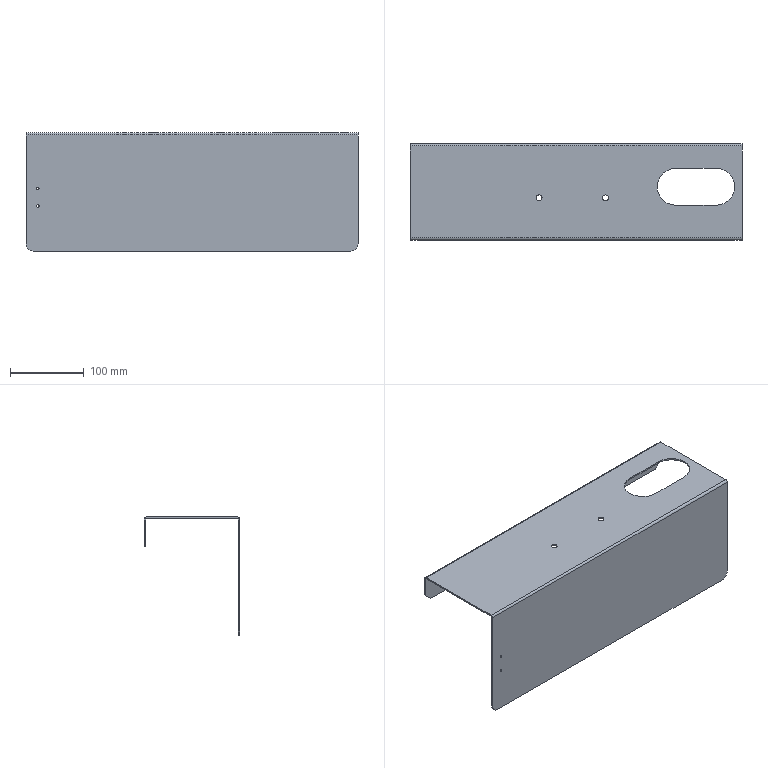Component | SolidWorks | -LowerGuard-1 | 1 solid | 39 faces | box 450 x 130 x 160 mm | volume 282110 mm3 | plane 22 | cylinder 17 | commonest cylinder face diameters 3.3 x4 8 x4 50 x3 5.473 x2 1.473 x2 20 x2
STEP:
#1=COLOUR_RGB('',0.7922,0.8196,0.9333);
#2=FILL_AREA_STYLE_COLOUR('',#1);
#3=FILL_AREA_STYLE('',(#2));
#4=SURFACE_STYLE_FILL_AREA(#3);
#5=SURFACE_SIDE_STYLE('',(#4));
#6=SURFACE_STYLE_USAGE(.BOTH.,#5);
#7=PRESENTATION_STYLE_ASSIGNMENT((#6));
#8=CARTESIAN_POINT('',(9.843,43.091,6.89));
#9=VERTEX_POINT('',#8);
#10=CARTESIAN_POINT('',(8.858,44.075,6.89));
#11=VERTEX_POINT('',#10);
#12=CARTESIAN_POINT('',(8.858,43.091,6.89));
#13=DIRECTION('',(-0.,0.,1.));
#14=DIRECTION('',(1.,0.,0.));
#15=AXIS2_PLACEMENT_3D('',#12,#13,#14);
#16=CIRCLE('',#15,0.9843);
#17=EDGE_CURVE('',#9,#11,#16,.T.);
#18=ORIENTED_EDGE('',*,*,#17,.F.);
#19=CARTESIAN_POINT('',(9.843,43.091,6.969));
#20=VERTEX_POINT('',#19);
#21=CARTESIAN_POINT('',(9.843,43.091,0.6693));
#22=DIRECTION('',(-0.,0.,1.));
#23=VECTOR('',#22,39.37);
#24=LINE('',#21,#23);
#25=EDGE_CURVE('',#9,#20,#24,.T.);
#26=ORIENTED_EDGE('',*,*,#25,.T.);
#27=CARTESIAN_POINT('',(8.858,44.075,6.969));
#28=VERTEX_POINT('',#27);
#29=CARTESIAN_POINT('',(8.858,43.091,6.969));
#30=DIRECTION('',(-0.,0.,1.));
#31=DIRECTION('',(1.,0.,0.));
#32=AXIS2_PLACEMENT_3D('',#29,#30,#31);
#33=CIRCLE('',#32,0.9843);
#34=EDGE_CURVE('',#20,#28,#33,.T.);
#35=ORIENTED_EDGE('',*,*,#34,.T.);
#36=CARTESIAN_POINT('',(8.858,44.075,0.6693));
#37=DIRECTION('',(-0.,0.,1.));
#38=VECTOR('',#37,39.37);
#39=LINE('',#36,#38);
#40=EDGE_CURVE('',#11,#28,#39,.T.);
#41=ORIENTED_EDGE('',*,*,#40,.F.);
#42=EDGE_LOOP('',(#18,#26,#35,#41));
#43=FACE_OUTER_BOUND('',#42,.T.);
#44=CARTESIAN_POINT('',(8.858,43.091,0.6693));
#45=DIRECTION('',(-0.,0.,1.));
#46=DIRECTION('',(1.,0.,0.));
#47=AXIS2_PLACEMENT_3D('',#44,#45,#46);
#48=CYLINDRICAL_SURFACE('',#47,0.9843);
#49=ADVANCED_FACE('',(#43),#48,.F.);
#50=CARTESIAN_POINT('',(-6.85,40.256,4.081));
#51=VERTEX_POINT('',#50);
#52=CARTESIAN_POINT('',(-6.85,40.256,3.951));
#53=VERTEX_POINT('',#52);
#54=CARTESIAN_POINT('',(-6.85,40.256,4.016));
#55=DIRECTION('',(-0.,1.,-0.));
#56=DIRECTION('',(0.,0.,-1.));
#57=AXIS2_PLACEMENT_3D('',#54,#55,#56);
#58=CIRCLE('',#57,0.06496);
#59=EDGE_CURVE('',#51,#53,#58,.T.);
#60=ORIENTED_EDGE('',*,*,#59,.F.);
#61=CARTESIAN_POINT('',(-6.85,40.335,4.081));
#62=VERTEX_POINT('',#61);
#63=CARTESIAN_POINT('',(-6.85,40.335,4.081));
#64=DIRECTION('',(-0.,1.,-0.));
#65=VECTOR('',#64,39.37);
#66=LINE('',#63,#65);
#67=EDGE_CURVE('',#51,#62,#66,.T.);
#68=ORIENTED_EDGE('',*,*,#67,.T.);
#69=CARTESIAN_POINT('',(-6.85,40.335,3.951));
#70=VERTEX_POINT('',#69);
#71=CARTESIAN_POINT('',(-6.85,40.335,4.016));
#72=DIRECTION('',(-0.,1.,-0.));
#73=DIRECTION('',(0.,0.,-1.));
#74=AXIS2_PLACEMENT_3D('',#71,#72,#73);
#75=CIRCLE('',#74,0.06496);
#76=EDGE_CURVE('',#62,#70,#75,.T.);
#77=ORIENTED_EDGE('',*,*,#76,.T.);
#78=CARTESIAN_POINT('',(-6.85,40.335,3.951));
#79=DIRECTION('',(-0.,1.,-0.));
#80=VECTOR('',#79,39.37);
#81=LINE('',#78,#80);
#82=EDGE_CURVE('',#53,#70,#81,.T.);
#83=ORIENTED_EDGE('',*,*,#82,.F.);
#84=EDGE_LOOP('',(#60,#68,#77,#83));
#85=FACE_OUTER_BOUND('',#84,.T.);
#86=CARTESIAN_POINT('',(-6.85,40.335,4.016));
#87=DIRECTION('',(-0.,1.,-0.));
#88=DIRECTION('',(0.,0.,-1.));
#89=AXIS2_PLACEMENT_3D('',#86,#87,#88);
#90=CYLINDRICAL_SURFACE('',#89,0.06496);
#91=ADVANCED_FACE('',(#85),#90,.F.);
#92=CARTESIAN_POINT('',(-6.85,40.256,3.136));
#93=VERTEX_POINT('',#92);
#94=CARTESIAN_POINT('',(-6.85,40.256,3.006));
#95=VERTEX_POINT('',#94);
#96=CARTESIAN_POINT('',(-6.85,40.256,3.071));
#97=DIRECTION('',(-0.,1.,-0.));
#98=DIRECTION('',(0.,0.,-1.));
#99=AXIS2_PLACEMENT_3D('',#96,#97,#98);
#100=CIRCLE('',#99,0.06496);
#101=EDGE_CURVE('',#93,#95,#100,.T.);
#102=ORIENTED_EDGE('',*,*,#101,.F.);
#103=CARTESIAN_POINT('',(-6.85,40.335,3.136));
#104=VERTEX_POINT('',#103);
#105=CARTESIAN_POINT('',(-6.85,40.335,3.136));
#106=DIRECTION('',(-0.,1.,-0.));
#107=VECTOR('',#106,39.37);
#108=LINE('',#105,#107);
#109=EDGE_CURVE('',#93,#104,#108,.T.);
#110=ORIENTED_EDGE('',*,*,#109,.T.);
#111=CARTESIAN_POINT('',(-6.85,40.335,3.006));
#112=VERTEX_POINT('',#111);
#113=CARTESIAN_POINT('',(-6.85,40.335,3.071));
#114=DIRECTION('',(-0.,1.,-0.));
#115=DIRECTION('',(0.,0.,-1.));
#116=AXIS2_PLACEMENT_3D('',#113,#114,#115);
#117=CIRCLE('',#116,0.06496);
#118=EDGE_CURVE('',#104,#112,#117,.T.);
#119=ORIENTED_EDGE('',*,*,#118,.T.);
#120=CARTESIAN_POINT('',(-6.85,40.335,3.006));
#121=DIRECTION('',(-0.,1.,-0.));
#122=VECTOR('',#121,39.37);
#123=LINE('',#120,#122);
#124=EDGE_CURVE('',#95,#112,#123,.T.);
#125=ORIENTED_EDGE('',*,*,#124,.F.);
#126=EDGE_LOOP('',(#102,#110,#119,#125));
#127=FACE_OUTER_BOUND('',#126,.T.);
#128=CARTESIAN_POINT('',(-6.85,40.335,3.071));
#129=DIRECTION('',(-0.,1.,-0.));
#130=DIRECTION('',(0.,0.,-1.));
#131=AXIS2_PLACEMENT_3D('',#128,#129,#130);
#132=CYLINDRICAL_SURFACE('',#131,0.06496);
#133=ADVANCED_FACE('',(#127),#132,.F.);
#134=CARTESIAN_POINT('',(2.795,42.5,6.89));
#135=VERTEX_POINT('',#134);
#136=CARTESIAN_POINT('',(3.11,42.5,6.89));
#137=VERTEX_POINT('',#136);
#138=CARTESIAN_POINT('',(2.953,42.5,6.89));
#139=DIRECTION('',(-0.,0.,1.));
#140=DIRECTION('',(1.,0.,0.));
#141=AXIS2_PLACEMENT_3D('',#138,#139,#140);
#142=CIRCLE('',#141,0.1575);
#143=EDGE_CURVE('',#135,#137,#142,.T.);
#144=ORIENTED_EDGE('',*,*,#143,.F.);
#145=CARTESIAN_POINT('',(2.795,42.5,6.969));
#146=VERTEX_POINT('',#145);
#147=CARTESIAN_POINT('',(2.795,42.5,6.575));
#148=DIRECTION('',(-0.,0.,1.));
#149=VECTOR('',#148,39.37);
#150=LINE('',#147,#149);
#151=EDGE_CURVE('',#135,#146,#150,.T.);
#152=ORIENTED_EDGE('',*,*,#151,.T.);
#153=CARTESIAN_POINT('',(3.11,42.5,6.969));
#154=VERTEX_POINT('',#153);
#155=CARTESIAN_POINT('',(2.953,42.5,6.969));
#156=DIRECTION('',(-0.,0.,1.));
#157=DIRECTION('',(1.,0.,0.));
#158=AXIS2_PLACEMENT_3D('',#155,#156,#157);
#159=CIRCLE('',#158,0.1575);
#160=EDGE_CURVE('',#146,#154,#159,.T.);
#161=ORIENTED_EDGE('',*,*,#160,.T.);
#162=CARTESIAN_POINT('',(3.11,42.5,6.575));
#163=DIRECTION('',(-0.,0.,1.));
#164=VECTOR('',#163,39.37);
#165=LINE('',#162,#164);
#166=EDGE_CURVE('',#137,#154,#165,.T.);
#167=ORIENTED_EDGE('',*,*,#166,.F.);
#168=EDGE_LOOP('',(#144,#152,#161,#167));
#169=FACE_OUTER_BOUND('',#168,.T.);
#170=CARTESIAN_POINT('',(2.953,42.5,6.575));
#171=DIRECTION('',(-0.,0.,1.));
#172=DIRECTION('',(1.,0.,0.));
#173=AXIS2_PLACEMENT_3D('',#170,#171,#172);
#174=CYLINDRICAL_SURFACE('',#173,0.1575);
#175=ADVANCED_FACE('',(#169),#174,.F.);
#176=CARTESIAN_POINT('',(-0.748,42.5,6.89));
#177=VERTEX_POINT('',#176);
#178=CARTESIAN_POINT('',(-0.4331,42.5,6.89));
#179=VERTEX_POINT('',#178);
#180=CARTESIAN_POINT('',(-0.5906,42.5,6.89));
#181=DIRECTION('',(-0.,0.,1.));
#182=DIRECTION('',(1.,0.,0.));
#183=AXIS2_PLACEMENT_3D('',#180,#181,#182);
#184=CIRCLE('',#183,0.1575);
#185=EDGE_CURVE('',#177,#179,#184,.T.);
#186=ORIENTED_EDGE('',*,*,#185,.F.);
#187=CARTESIAN_POINT('',(-0.748,42.5,6.969));
#188=VERTEX_POINT('',#187);
#189=CARTESIAN_POINT('',(-0.748,42.5,6.575));
#190=DIRECTION('',(-0.,0.,1.));
#191=VECTOR('',#190,39.37);
#192=LINE('',#189,#191);
#193=EDGE_CURVE('',#177,#188,#192,.T.);
#194=ORIENTED_EDGE('',*,*,#193,.T.);
#195=CARTESIAN_POINT('',(-0.4331,42.5,6.969));
#196=VERTEX_POINT('',#195);
#197=CARTESIAN_POINT('',(-0.5906,42.5,6.969));
#198=DIRECTION('',(-0.,0.,1.));
#199=DIRECTION('',(1.,0.,0.));
#200=AXIS2_PLACEMENT_3D('',#197,#198,#199);
#201=CIRCLE('',#200,0.1575);
#202=EDGE_CURVE('',#188,#196,#201,.T.);
#203=ORIENTED_EDGE('',*,*,#202,.T.);
#204=CARTESIAN_POINT('',(-0.4331,42.5,6.575));
#205=DIRECTION('',(-0.,0.,1.));
#206=VECTOR('',#205,39.37);
#207=LINE('',#204,#206);
#208=EDGE_CURVE('',#179,#196,#207,.T.);
#209=ORIENTED_EDGE('',*,*,#208,.F.);
#210=EDGE_LOOP('',(#186,#194,#203,#209));
#211=FACE_OUTER_BOUND('',#210,.T.);
#212=CARTESIAN_POINT('',(-0.5906,42.5,6.575));
#213=DIRECTION('',(-0.,0.,1.));
#214=DIRECTION('',(1.,0.,0.));
#215=AXIS2_PLACEMENT_3D('',#212,#213,#214);
#216=CYLINDRICAL_SURFACE('',#215,0.1575);
#217=ADVANCED_FACE('',(#211),#216,.F.);
#218=CARTESIAN_POINT('',(-7.48,40.256,6.861));
#219=VERTEX_POINT('',#218);
#220=CARTESIAN_POINT('',(-7.48,40.335,6.861));
#221=VERTEX_POINT('',#220);
#222=CARTESIAN_POINT('',(-7.48,40.256,6.861));
#223=DIRECTION('',(-0.,1.,-0.));
#224=VECTOR('',#223,39.37);
#225=LINE('',#222,#224);
#226=EDGE_CURVE('',#219,#221,#225,.T.);
#227=ORIENTED_EDGE('',*,*,#226,.F.);
#228=CARTESIAN_POINT('',(-7.48,40.364,6.969));
#229=VERTEX_POINT('',#228);
#230=CARTESIAN_POINT('',(-7.48,40.364,6.861));
#231=DIRECTION('',(1.,0.,0.));
#232=DIRECTION('',(0.,0.,1.));
#233=AXIS2_PLACEMENT_3D('',#230,#231,#232);
#234=CIRCLE('',#233,0.1077);
#235=EDGE_CURVE('',#229,#219,#234,.T.);
#236=ORIENTED_EDGE('',*,*,#235,.F.);
#237=CARTESIAN_POINT('',(-7.48,40.364,6.89));
#238=VERTEX_POINT('',#237);
#239=CARTESIAN_POINT('',(-7.48,40.364,6.89));
#240=DIRECTION('',(-0.,0.,1.));
#241=VECTOR('',#240,39.37);
#242=LINE('',#239,#241);
#243=EDGE_CURVE('',#238,#229,#242,.T.);
#244=ORIENTED_EDGE('',*,*,#243,.F.);
#245=CARTESIAN_POINT('',(-7.48,40.364,6.861));
#246=DIRECTION('',(1.,0.,0.));
#247=DIRECTION('',(0.,0.,1.));
#248=AXIS2_PLACEMENT_3D('',#245,#246,#247);
#249=CIRCLE('',#248,0.029);
#250=EDGE_CURVE('',#238,#221,#249,.T.);
#251=ORIENTED_EDGE('',*,*,#250,.T.);
#252=EDGE_LOOP('',(#227,#236,#244,#251));
#253=FACE_OUTER_BOUND('',#252,.T.);
#254=CARTESIAN_POINT('',(-7.48,40.256,6.861));
#255=DIRECTION('',(-1.,-0.,-0.));
#256=DIRECTION('',(-0.,0.,1.));
#257=AXIS2_PLACEMENT_3D('',#254,#255,#256);
#258=PLANE('',#257);
#259=ADVANCED_FACE('',(#253),#258,.T.);
#260=CARTESIAN_POINT('',(-7.48,40.335,1.063));
#261=VERTEX_POINT('',#260);
#262=CARTESIAN_POINT('',(-7.48,40.335,6.969));
#263=DIRECTION('',(0.,-0.,-1.));
#264=VECTOR('',#263,39.37);
#265=LINE('',#262,#264);
#266=EDGE_CURVE('',#221,#261,#265,.T.);
#267=ORIENTED_EDGE('',*,*,#266,.T.);
#268=CARTESIAN_POINT('',(-7.48,40.256,1.063));
#269=VERTEX_POINT('',#268);
#270=CARTESIAN_POINT('',(-7.48,40.364,1.063));
#271=DIRECTION('',(0.,-1.,0.));
#272=VECTOR('',#271,39.37);
#273=LINE('',#270,#272);
#274=EDGE_CURVE('',#261,#269,#273,.T.);
#275=ORIENTED_EDGE('',*,*,#274,.T.);
#276=CARTESIAN_POINT('',(-7.48,40.256,6.969));
#277=DIRECTION('',(0.,-0.,-1.));
#278=VECTOR('',#277,39.37);
#279=LINE('',#276,#278);
#280=EDGE_CURVE('',#219,#269,#279,.T.);
#281=ORIENTED_EDGE('',*,*,#280,.F.);
#282=ORIENTED_EDGE('',*,*,#226,.T.);
#283=EDGE_LOOP('',(#267,#275,#281,#282));
#284=FACE_OUTER_BOUND('',#283,.T.);
#285=CARTESIAN_POINT('',(-7.48,40.364,6.89));
#286=DIRECTION('',(-1.,-0.,-0.));
#287=DIRECTION('',(-0.,0.,1.));
#288=AXIS2_PLACEMENT_3D('',#285,#286,#287);
#289=PLANE('',#288);
#290=ADVANCED_FACE('',(#284),#289,.T.);
#291=CARTESIAN_POINT('',(10.236,40.364,6.969));
#292=VERTEX_POINT('',#291);
#293=CARTESIAN_POINT('',(10.236,40.364,6.89));
#294=VERTEX_POINT('',#293);
#295=CARTESIAN_POINT('',(10.236,40.364,6.969));
#296=DIRECTION('',(0.,-0.,-1.));
#297=VECTOR('',#296,39.37);
#298=LINE('',#295,#297);
#299=EDGE_CURVE('',#292,#294,#298,.T.);
#300=ORIENTED_EDGE('',*,*,#299,.F.);
#301=CARTESIAN_POINT('',(10.236,40.256,6.861));
#302=VERTEX_POINT('',#301);
#303=CARTESIAN_POINT('',(10.236,40.364,6.861));
#304=DIRECTION('',(1.,0.,0.));
#305=DIRECTION('',(0.,0.,1.));
#306=AXIS2_PLACEMENT_3D('',#303,#304,#305);
#307=CIRCLE('',#306,0.1077);
#308=EDGE_CURVE('',#292,#302,#307,.T.);
#309=ORIENTED_EDGE('',*,*,#308,.T.);
#310=CARTESIAN_POINT('',(10.236,40.335,6.861));
#311=VERTEX_POINT('',#310);
#312=CARTESIAN_POINT('',(10.236,40.335,6.861));
#313=DIRECTION('',(0.,-1.,0.));
#314=VECTOR('',#313,39.37);
#315=LINE('',#312,#314);
#316=EDGE_CURVE('',#311,#302,#315,.T.);
#317=ORIENTED_EDGE('',*,*,#316,.F.);
#318=CARTESIAN_POINT('',(10.236,40.364,6.861));
#319=DIRECTION('',(1.,0.,0.));
#320=DIRECTION('',(0.,0.,1.));
#321=AXIS2_PLACEMENT_3D('',#318,#319,#320);
#322=CIRCLE('',#321,0.029);
#323=EDGE_CURVE('',#294,#311,#322,.T.);
#324=ORIENTED_EDGE('',*,*,#323,.F.);
#325=EDGE_LOOP('',(#300,#309,#317,#324));
#326=FACE_OUTER_BOUND('',#325,.T.);
#327=CARTESIAN_POINT('',(10.236,40.364,6.969));
#328=DIRECTION('',(1.,0.,0.));
#329=DIRECTION('',(0.,-0.,-1.));
#330=AXIS2_PLACEMENT_3D('',#327,#328,#329);
#331=PLANE('',#330);
#332=ADVANCED_FACE('',(#326),#331,.T.);
#333=CARTESIAN_POINT('',(10.236,45.266,6.969));
#334=VERTEX_POINT('',#333);
#335=CARTESIAN_POINT('',(10.236,45.177,6.969));
#336=DIRECTION('',(0.,-1.,0.));
#337=VECTOR('',#336,39.37);
#338=LINE('',#335,#337);
#339=EDGE_CURVE('',#334,#292,#338,.T.);
#340=ORIENTED_EDGE('',*,*,#339,.T.);
#341=ORIENTED_EDGE('',*,*,#299,.T.);
#342=CARTESIAN_POINT('',(10.236,45.266,6.89));
#343=VERTEX_POINT('',#342);
#344=CARTESIAN_POINT('',(10.236,45.177,6.89));
#345=DIRECTION('',(0.,-1.,0.));
#346=VECTOR('',#345,39.37);
#347=LINE('',#344,#346);
#348=EDGE_CURVE('',#343,#294,#347,.T.);
#349=ORIENTED_EDGE('',*,*,#348,.F.);
#350=CARTESIAN_POINT('',(10.236,45.266,6.89));
#351=DIRECTION('',(-0.,0.,1.));
#352=VECTOR('',#351,39.37);
#353=LINE('',#350,#352);
#354=EDGE_CURVE('',#343,#334,#353,.T.);
#355=ORIENTED_EDGE('',*,*,#354,.T.);
#356=EDGE_LOOP('',(#340,#341,#349,#355));
#357=FACE_OUTER_BOUND('',#356,.T.);
#358=CARTESIAN_POINT('',(10.236,40.335,6.861));
#359=DIRECTION('',(1.,0.,0.));
#360=DIRECTION('',(0.,-0.,-1.));
#361=AXIS2_PLACEMENT_3D('',#358,#359,#360);
#362=PLANE('',#361);
#363=ADVANCED_FACE('',(#357),#362,.T.);
#364=CARTESIAN_POINT('',(-6.85,40.335,4.016));
#365=DIRECTION('',(-0.,1.,-0.));
#366=DIRECTION('',(0.,0.,-1.));
#367=AXIS2_PLACEMENT_3D('',#364,#365,#366);
#368=CIRCLE('',#367,0.06496);
#369=EDGE_CURVE('',#70,#62,#368,.T.);
#370=ORIENTED_EDGE('',*,*,#369,.F.);
#371=ORIENTED_EDGE('',*,*,#76,.F.);
#372=EDGE_LOOP('',(#370,#371));
#373=FACE_BOUND('',#372,.T.);
#374=CARTESIAN_POINT('',(-6.85,40.335,3.071));
#375=DIRECTION('',(-0.,1.,-0.));
#376=DIRECTION('',(0.,0.,-1.));
#377=AXIS2_PLACEMENT_3D('',#374,#375,#376);
#378=CIRCLE('',#377,0.06496);
#379=EDGE_CURVE('',#112,#104,#378,.T.);
#380=ORIENTED_EDGE('',*,*,#379,.F.);
#381=ORIENTED_EDGE('',*,*,#118,.F.);
#382=EDGE_LOOP('',(#380,#381));
#383=FACE_BOUND('',#382,.T.);
#384=CARTESIAN_POINT('',(-7.087,40.335,0.6693));
#385=VERTEX_POINT('',#384);
#386=CARTESIAN_POINT('',(9.843,40.335,0.6693));
#387=VERTEX_POINT('',#386);
#388=CARTESIAN_POINT('',(-7.48,40.335,0.6693));
#389=DIRECTION('',(1.,0.,0.));
#390=VECTOR('',#389,39.37);
#391=LINE('',#388,#390);
#392=EDGE_CURVE('',#385,#387,#391,.T.);
#393=ORIENTED_EDGE('',*,*,#392,.F.);
#394=CARTESIAN_POINT('',(-7.087,40.335,1.063));
#395=DIRECTION('',(-0.,1.,-0.));
#396=DIRECTION('',(0.,0.,1.));
#397=AXIS2_PLACEMENT_3D('',#394,#395,#396);
#398=CIRCLE('',#397,0.3937);
#399=EDGE_CURVE('',#385,#261,#398,.T.);
#400=ORIENTED_EDGE('',*,*,#399,.T.);
#401=ORIENTED_EDGE('',*,*,#266,.F.);
#402=CARTESIAN_POINT('',(-7.48,40.335,6.861));
#403=DIRECTION('',(1.,0.,0.));
#404=VECTOR('',#403,39.37);
#405=LINE('',#402,#404);
#406=EDGE_CURVE('',#221,#311,#405,.T.);
#407=ORIENTED_EDGE('',*,*,#406,.T.);
#408=CARTESIAN_POINT('',(10.236,40.335,1.063));
#409=VERTEX_POINT('',#408);
#410=CARTESIAN_POINT('',(10.236,40.335,6.969));
#411=DIRECTION('',(0.,-0.,-1.));
#412=VECTOR('',#411,39.37);
#413=LINE('',#410,#412);
#414=EDGE_CURVE('',#311,#409,#413,.T.);
#415=ORIENTED_EDGE('',*,*,#414,.T.);
#416=CARTESIAN_POINT('',(9.843,40.335,1.063));
#417=DIRECTION('',(-0.,1.,-0.));
#418=DIRECTION('',(0.,0.,1.));
#419=AXIS2_PLACEMENT_3D('',#416,#417,#418);
#420=CIRCLE('',#419,0.3937);
#421=EDGE_CURVE('',#409,#387,#420,.T.);
#422=ORIENTED_EDGE('',*,*,#421,.T.);
#423=EDGE_LOOP('',(#393,#400,#401,#407,#415,#422));
#424=FACE_OUTER_BOUND('',#423,.T.);
#425=CARTESIAN_POINT('',(-7.48,40.335,6.969));
#426=DIRECTION('',(0.,-1.,0.));
#427=DIRECTION('',(-0.,0.,1.));
#428=AXIS2_PLACEMENT_3D('',#425,#426,#427);
#429=PLANE('',#428);
#430=ADVANCED_FACE('',(#373,#383,#424),#429,.F.);
#431=CARTESIAN_POINT('',(-7.087,40.256,0.6693));
#432=VERTEX_POINT('',#431);
#433=CARTESIAN_POINT('',(9.843,40.256,0.6693));
#434=VERTEX_POINT('',#433);
#435=CARTESIAN_POINT('',(-7.48,40.256,0.6693));
#436=DIRECTION('',(1.,0.,0.));
#437=VECTOR('',#436,39.37);
#438=LINE('',#435,#437);
#439=EDGE_CURVE('',#432,#434,#438,.T.);
#440=ORIENTED_EDGE('',*,*,#439,.F.);
#441=CARTESIAN_POINT('',(-7.087,40.256,0.6693));
#442=DIRECTION('',(-0.,1.,-0.));
#443=VECTOR('',#442,39.37);
#444=LINE('',#441,#443);
#445=EDGE_CURVE('',#432,#385,#444,.T.);
#446=ORIENTED_EDGE('',*,*,#445,.T.);
#447=ORIENTED_EDGE('',*,*,#392,.T.);
#448=CARTESIAN_POINT('',(9.843,40.256,0.6693));
#449=DIRECTION('',(0.,-1.,0.));
#450=VECTOR('',#449,39.37);
#451=LINE('',#448,#450);
#452=EDGE_CURVE('',#387,#434,#451,.T.);
#453=ORIENTED_EDGE('',*,*,#452,.T.);
#454=EDGE_LOOP('',(#440,#446,#447,#453));
#455=FACE_OUTER_BOUND('',#454,.T.);
#456=CARTESIAN_POINT('',(-7.48,40.256,0.6693));
#457=DIRECTION('',(0.,-0.,-1.));
#458=DIRECTION('',(-1.,-0.,-0.));
#459=AXIS2_PLACEMENT_3D('',#456,#457,#458);
#460=PLANE('',#459);
#461=ADVANCED_FACE('',(#455),#460,.T.);
#462=CARTESIAN_POINT('',(-6.85,40.256,4.016));
#463=DIRECTION('',(-0.,1.,-0.));
#464=DIRECTION('',(0.,0.,-1.));
#465=AXIS2_PLACEMENT_3D('',#462,#463,#464);
#466=CIRCLE('',#465,0.06496);
#467=EDGE_CURVE('',#53,#51,#466,.T.);
#468=ORIENTED_EDGE('',*,*,#467,.T.);
#469=ORIENTED_EDGE('',*,*,#59,.T.);
#470=EDGE_LOOP('',(#468,#469));
#471=FACE_BOUND('',#470,.T.);
#472=CARTESIAN_POINT('',(-6.85,40.256,3.071));
#473=DIRECTION('',(-0.,1.,-0.));
#474=DIRECTION('',(0.,0.,-1.));
#475=AXIS2_PLACEMENT_3D('',#472,#473,#474);
#476=CIRCLE('',#475,0.06496);
#477=EDGE_CURVE('',#95,#93,#476,.T.);
#478=ORIENTED_EDGE('',*,*,#477,.T.);
#479=ORIENTED_EDGE('',*,*,#101,.T.);
#480=EDGE_LOOP('',(#478,#479));
#481=FACE_BOUND('',#480,.T.);
#482=ORIENTED_EDGE('',*,*,#280,.T.);
#483=CARTESIAN_POINT('',(-7.087,40.256,1.063));
#484=DIRECTION('',(0.,-1.,0.));
#485=DIRECTION('',(0.,0.,1.));
#486=AXIS2_PLACEMENT_3D('',#483,#484,#485);
#487=CIRCLE('',#486,0.3937);
#488=EDGE_CURVE('',#269,#432,#487,.T.);
#489=ORIENTED_EDGE('',*,*,#488,.T.);
#490=ORIENTED_EDGE('',*,*,#439,.T.);
#491=CARTESIAN_POINT('',(10.236,40.256,1.063));
#492=VERTEX_POINT('',#491);
#493=CARTESIAN_POINT('',(9.843,40.256,1.063));
#494=DIRECTION('',(0.,-1.,0.));
#495=DIRECTION('',(0.,0.,1.));
#496=AXIS2_PLACEMENT_3D('',#493,#494,#495);
#497=CIRCLE('',#496,0.3937);
#498=EDGE_CURVE('',#434,#492,#497,.T.);
#499=ORIENTED_EDGE('',*,*,#498,.T.);
#500=CARTESIAN_POINT('',(10.236,40.256,6.969));
#501=DIRECTION('',(0.,-0.,-1.));
#502=VECTOR('',#501,39.37);
#503=LINE('',#500,#502);
#504=EDGE_CURVE('',#302,#492,#503,.T.);
#505=ORIENTED_EDGE('',*,*,#504,.F.);
#506=CARTESIAN_POINT('',(-7.48,40.256,6.861));
#507=DIRECTION('',(1.,0.,0.));
#508=VECTOR('',#507,39.37);
#509=LINE('',#506,#508);
#510=EDGE_CURVE('',#219,#302,#509,.T.);
#511=ORIENTED_EDGE('',*,*,#510,.F.);
#512=EDGE_LOOP('',(#482,#489,#490,#499,#505,#511));
#513=FACE_OUTER_BOUND('',#512,.T.);
#514=CARTESIAN_POINT('',(-7.48,40.256,6.969));
#515=DIRECTION('',(0.,-1.,0.));
#516=DIRECTION('',(-0.,0.,1.));
#517=AXIS2_PLACEMENT_3D('',#514,#515,#516);
#518=PLANE('',#517);
#519=ADVANCED_FACE('',(#471,#481,#513),#518,.T.);
#520=ORIENTED_EDGE('',*,*,#308,.F.);
#521=CARTESIAN_POINT('',(-7.48,40.364,6.969));
#522=DIRECTION('',(1.,0.,0.));
#523=VECTOR('',#522,39.37);
#524=LINE('',#521,#523);
#525=EDGE_CURVE('',#229,#292,#524,.T.);
#526=ORIENTED_EDGE('',*,*,#525,.F.);
#527=ORIENTED_EDGE('',*,*,#235,.T.);
#528=ORIENTED_EDGE('',*,*,#510,.T.);
#529=EDGE_LOOP('',(#520,#526,#527,#528));
#530=FACE_OUTER_BOUND('',#529,.T.);
#531=CARTESIAN_POINT('',(-7.48,40.364,6.861));
#532=DIRECTION('',(1.,0.,0.));
#533=DIRECTION('',(0.,0.,-1.));
#534=AXIS2_PLACEMENT_3D('',#531,#532,#533);
#535=CYLINDRICAL_SURFACE('',#534,0.1077);
#536=ADVANCED_FACE('',(#530),#535,.T.);
#537=CARTESIAN_POINT('',(6.693,44.075,6.969));
#538=VERTEX_POINT('',#537);
#539=CARTESIAN_POINT('',(6.693,42.106,6.969));
#540=VERTEX_POINT('',#539);
#541=CARTESIAN_POINT('',(6.693,43.091,6.969));
#542=DIRECTION('',(-0.,0.,1.));
#543=DIRECTION('',(1.,0.,0.));
#544=AXIS2_PLACEMENT_3D('',#541,#542,#543);
#545=CIRCLE('',#544,0.9843);
#546=EDGE_CURVE('',#538,#540,#545,.T.);
#547=ORIENTED_EDGE('',*,*,#546,.F.);
#548=CARTESIAN_POINT('',(6.693,44.075,6.969));
#549=DIRECTION('',(-1.,-0.,-0.));
#550=VECTOR('',#549,39.37);
#551=LINE('',#548,#550);
#552=EDGE_CURVE('',#28,#538,#551,.T.);
#553=ORIENTED_EDGE('',*,*,#552,.F.);
#554=ORIENTED_EDGE('',*,*,#34,.F.);
#555=CARTESIAN_POINT('',(8.858,42.106,6.969));
#556=VERTEX_POINT('',#555);
#557=CARTESIAN_POINT('',(8.858,43.091,6.969));
#558=DIRECTION('',(-0.,0.,1.));
#559=DIRECTION('',(1.,0.,0.));
#560=AXIS2_PLACEMENT_3D('',#557,#558,#559);
#561=CIRCLE('',#560,0.9843);
#562=EDGE_CURVE('',#556,#20,#561,.T.);
#563=ORIENTED_EDGE('',*,*,#562,.F.);
#564=CARTESIAN_POINT('',(6.693,42.106,6.969));
#565=DIRECTION('',(1.,0.,0.));
#566=VECTOR('',#565,39.37);
#567=LINE('',#564,#566);
#568=EDGE_CURVE('',#540,#556,#567,.T.);
#569=ORIENTED_EDGE('',*,*,#568,.F.);
#570=EDGE_LOOP('',(#547,#553,#554,#563,#569));
#571=FACE_BOUND('',#570,.T.);
#572=CARTESIAN_POINT('',(2.953,42.5,6.969));
#573=DIRECTION('',(-0.,0.,1.));
#574=DIRECTION('',(1.,0.,0.));
#575=AXIS2_PLACEMENT_3D('',#572,#573,#574);
#576=CIRCLE('',#575,0.1575);
#577=EDGE_CURVE('',#154,#146,#576,.T.);
#578=ORIENTED_EDGE('',*,*,#577,.F.);
#579=ORIENTED_EDGE('',*,*,#160,.F.);
#580=EDGE_LOOP('',(#578,#579));
#581=FACE_BOUND('',#580,.T.);
#582=CARTESIAN_POINT('',(-0.5906,42.5,6.969));
#583=DIRECTION('',(-0.,0.,1.));
#584=DIRECTION('',(1.,0.,0.));
#585=AXIS2_PLACEMENT_3D('',#582,#583,#584);
#586=CIRCLE('',#585,0.1575);
#587=EDGE_CURVE('',#196,#188,#586,.T.);
#588=ORIENTED_EDGE('',*,*,#587,.F.);
#589=ORIENTED_EDGE('',*,*,#202,.F.);
#590=EDGE_LOOP('',(#588,#589));
#591=FACE_BOUND('',#590,.T.);
#592=ORIENTED_EDGE('',*,*,#339,.F.);
#593=CARTESIAN_POINT('',(-7.48,45.266,6.969));
#594=VERTEX_POINT('',#593);
#595=CARTESIAN_POINT('',(10.236,45.266,6.969));
#596=DIRECTION('',(-1.,-0.,-0.));
#597=VECTOR('',#596,39.37);
#598=LINE('',#595,#597);
#599=EDGE_CURVE('',#334,#594,#598,.T.);
#600=ORIENTED_EDGE('',*,*,#599,.T.);
#601=CARTESIAN_POINT('',(-7.48,45.177,6.969));
#602=DIRECTION('',(0.,-1.,0.));
#603=VECTOR('',#602,39.37);
#604=LINE('',#601,#603);
#605=EDGE_CURVE('',#594,#229,#604,.T.);
#606=ORIENTED_EDGE('',*,*,#605,.T.);
#607=ORIENTED_EDGE('',*,*,#525,.T.);
#608=EDGE_LOOP('',(#592,#600,#606,#607));
#609=FACE_OUTER_BOUND('',#608,.T.);
#610=CARTESIAN_POINT('',(-7.48,45.177,6.969));
#611=DIRECTION('',(-0.,0.,1.));
#612=DIRECTION('',(1.,0.,0.));
#613=AXIS2_PLACEMENT_3D('',#610,#611,#612);
#614=PLANE('',#613);
#615=ADVANCED_FACE('',(#571,#581,#591,#609),#614,.T.);
#616=CARTESIAN_POINT('',(6.693,44.075,6.89));
#617=VERTEX_POINT('',#616);
#618=CARTESIAN_POINT('',(-7.48,44.075,6.89));
#619=DIRECTION('',(-1.,-0.,-0.));
#620=VECTOR('',#619,39.37);
#621=LINE('',#618,#620);
#622=EDGE_CURVE('',#11,#617,#621,.T.);
#623=ORIENTED_EDGE('',*,*,#622,.T.);
#624=CARTESIAN_POINT('',(6.693,42.106,6.89));
#625=VERTEX_POINT('',#624);
#626=CARTESIAN_POINT('',(6.693,43.091,6.89));
#627=DIRECTION('',(-0.,0.,1.));
#628=DIRECTION('',(1.,0.,0.));
#629=AXIS2_PLACEMENT_3D('',#626,#627,#628);
#630=CIRCLE('',#629,0.9843);
#631=EDGE_CURVE('',#617,#625,#630,.T.);
#632=ORIENTED_EDGE('',*,*,#631,.T.);
#633=CARTESIAN_POINT('',(8.858,42.106,6.89));
#634=VERTEX_POINT('',#633);
#635=CARTESIAN_POINT('',(-7.48,42.106,6.89));
#636=DIRECTION('',(1.,0.,0.));
#637=VECTOR('',#636,39.37);
#638=LINE('',#635,#637);
#639=EDGE_CURVE('',#625,#634,#638,.T.);
#640=ORIENTED_EDGE('',*,*,#639,.T.);
#641=CARTESIAN_POINT('',(8.858,43.091,6.89));
#642=DIRECTION('',(-0.,0.,1.));
#643=DIRECTION('',(1.,0.,0.));
#644=AXIS2_PLACEMENT_3D('',#641,#642,#643);
#645=CIRCLE('',#644,0.9843);
#646=EDGE_CURVE('',#634,#9,#645,.T.);
#647=ORIENTED_EDGE('',*,*,#646,.T.);
#648=ORIENTED_EDGE('',*,*,#17,.T.);
#649=EDGE_LOOP('',(#623,#632,#640,#647,#648));
#650=FACE_BOUND('',#649,.T.);
#651=CARTESIAN_POINT('',(2.953,42.5,6.89));
#652=DIRECTION('',(-0.,0.,1.));
#653=DIRECTION('',(1.,0.,0.));
#654=AXIS2_PLACEMENT_3D('',#651,#652,#653);
#655=CIRCLE('',#654,0.1575);
#656=EDGE_CURVE('',#137,#135,#655,.T.);
#657=ORIENTED_EDGE('',*,*,#656,.T.);
#658=ORIENTED_EDGE('',*,*,#143,.T.);
#659=EDGE_LOOP('',(#657,#658));
#660=FACE_BOUND('',#659,.T.);
#661=CARTESIAN_POINT('',(-0.5906,42.5,6.89));
#662=DIRECTION('',(-0.,0.,1.));
#663=DIRECTION('',(1.,0.,0.));
#664=AXIS2_PLACEMENT_3D('',#661,#662,#663);
#665=CIRCLE('',#664,0.1575);
#666=EDGE_CURVE('',#179,#177,#665,.T.);
#667=ORIENTED_EDGE('',*,*,#666,.T.);
#668=ORIENTED_EDGE('',*,*,#185,.T.);
#669=EDGE_LOOP('',(#667,#668));
#670=FACE_BOUND('',#669,.T.);
#671=ORIENTED_EDGE('',*,*,#348,.T.);
#672=CARTESIAN_POINT('',(-7.48,40.364,6.89));
#673=DIRECTION('',(1.,0.,0.));
#674=VECTOR('',#673,39.37);
#675=LINE('',#672,#674);
#676=EDGE_CURVE('',#238,#294,#675,.T.);
#677=ORIENTED_EDGE('',*,*,#676,.F.);
#678=CARTESIAN_POINT('',(-7.48,45.266,6.89));
#679=VERTEX_POINT('',#678);
#680=CARTESIAN_POINT('',(-7.48,45.177,6.89));
#681=DIRECTION('',(0.,-1.,0.));
#682=VECTOR('',#681,39.37);
#683=LINE('',#680,#682);
#684=EDGE_CURVE('',#679,#238,#683,.T.);
#685=ORIENTED_EDGE('',*,*,#684,.F.);
#686=CARTESIAN_POINT('',(10.236,45.266,6.89));
#687=DIRECTION('',(-1.,-0.,-0.));
#688=VECTOR('',#687,39.37);
#689=LINE('',#686,#688);
#690=EDGE_CURVE('',#343,#679,#689,.T.);
#691=ORIENTED_EDGE('',*,*,#690,.F.);
#692=EDGE_LOOP('',(#671,#677,#685,#691));
#693=FACE_OUTER_BOUND('',#692,.T.);
#694=CARTESIAN_POINT('',(-7.48,45.177,6.89));
#695=DIRECTION('',(-0.,0.,1.));
#696=DIRECTION('',(1.,0.,0.));
#697=AXIS2_PLACEMENT_3D('',#694,#695,#696);
#698=PLANE('',#697);
#699=ADVANCED_FACE('',(#650,#660,#670,#693),#698,.F.);
#700=ORIENTED_EDGE('',*,*,#323,.T.);
#701=ORIENTED_EDGE('',*,*,#406,.F.);
#702=ORIENTED_EDGE('',*,*,#250,.F.);
#703=ORIENTED_EDGE('',*,*,#676,.T.);
#704=EDGE_LOOP('',(#700,#701,#702,#703));
#705=FACE_OUTER_BOUND('',#704,.T.);
#706=CARTESIAN_POINT('',(-7.48,40.364,6.861));
#707=DIRECTION('',(1.,0.,0.));
#708=DIRECTION('',(0.,0.,-1.));
#709=AXIS2_PLACEMENT_3D('',#706,#707,#708);
#710=CYLINDRICAL_SURFACE('',#709,0.029);
#711=ADVANCED_FACE('',(#705),#710,.F.);
#712=ORIENTED_EDGE('',*,*,#684,.T.);
#713=ORIENTED_EDGE('',*,*,#243,.T.);
#714=ORIENTED_EDGE('',*,*,#605,.F.);
#715=CARTESIAN_POINT('',(-7.48,45.266,6.89));
#716=DIRECTION('',(-0.,0.,1.));
#717=VECTOR('',#716,39.37);
#718=LINE('',#715,#717);
#719=EDGE_CURVE('',#679,#594,#718,.T.);
#720=ORIENTED_EDGE('',*,*,#719,.F.);
#721=EDGE_LOOP('',(#712,#713,#714,#720));
#722=FACE_OUTER_BOUND('',#721,.T.);
#723=CARTESIAN_POINT('',(-7.48,40.364,6.861));
#724=DIRECTION('',(-1.,-0.,-0.));
#725=DIRECTION('',(-0.,0.,1.));
#726=AXIS2_PLACEMENT_3D('',#723,#724,#725);
#727=PLANE('',#726);
#728=ADVANCED_FACE('',(#722),#727,.T.);
#729=ORIENTED_EDGE('',*,*,#504,.T.);
#730=CARTESIAN_POINT('',(10.236,40.335,1.063));
#731=DIRECTION('',(-0.,1.,-0.));
#732=VECTOR('',#731,39.37);
#733=LINE('',#730,#732);
#734=EDGE_CURVE('',#492,#409,#733,.T.);
#735=ORIENTED_EDGE('',*,*,#734,.T.);
#736=ORIENTED_EDGE('',*,*,#414,.F.);
#737=ORIENTED_EDGE('',*,*,#316,.T.);
#738=EDGE_LOOP('',(#729,#735,#736,#737));
#739=FACE_OUTER_BOUND('',#738,.T.);
#740=CARTESIAN_POINT('',(10.236,40.364,6.861));
#741=DIRECTION('',(-1.,-0.,-0.));
#742=DIRECTION('',(-0.,0.,1.));
#743=AXIS2_PLACEMENT_3D('',#740,#741,#742);
#744=PLANE('',#743);
#745=ADVANCED_FACE('',(#739),#744,.F.);
#746=ORIENTED_EDGE('',*,*,#193,.F.);
#747=ORIENTED_EDGE('',*,*,#666,.F.);
#748=ORIENTED_EDGE('',*,*,#208,.T.);
#749=ORIENTED_EDGE('',*,*,#587,.T.);
#750=EDGE_LOOP('',(#746,#747,#748,#749));
#751=FACE_OUTER_BOUND('',#750,.T.);
#752=CARTESIAN_POINT('',(-0.5906,42.5,6.575));
#753=DIRECTION('',(-0.,0.,1.));
#754=DIRECTION('',(1.,0.,0.));
#755=AXIS2_PLACEMENT_3D('',#752,#753,#754);
#756=CYLINDRICAL_SURFACE('',#755,0.1575);
#757=ADVANCED_FACE('',(#751),#756,.F.);
#758=ORIENTED_EDGE('',*,*,#151,.F.);
#759=ORIENTED_EDGE('',*,*,#656,.F.);
#760=ORIENTED_EDGE('',*,*,#166,.T.);
#761=ORIENTED_EDGE('',*,*,#577,.T.);
#762=EDGE_LOOP('',(#758,#759,#760,#761));
#763=FACE_OUTER_BOUND('',#762,.T.);
#764=CARTESIAN_POINT('',(2.953,42.5,6.575));
#765=DIRECTION('',(-0.,0.,1.));
#766=DIRECTION('',(1.,0.,0.));
#767=AXIS2_PLACEMENT_3D('',#764,#765,#766);
#768=CYLINDRICAL_SURFACE('',#767,0.1575);
#769=ADVANCED_FACE('',(#763),#768,.F.);
#770=ORIENTED_EDGE('',*,*,#488,.F.);
#771=ORIENTED_EDGE('',*,*,#274,.F.);
#772=ORIENTED_EDGE('',*,*,#399,.F.);
#773=ORIENTED_EDGE('',*,*,#445,.F.);
#774=EDGE_LOOP('',(#770,#771,#772,#773));
#775=FACE_OUTER_BOUND('',#774,.T.);
#776=CARTESIAN_POINT('',(-7.087,40.256,1.063));
#777=DIRECTION('',(-0.,1.,-0.));
#778=DIRECTION('',(0.,0.,-1.));
#779=AXIS2_PLACEMENT_3D('',#776,#777,#778);
#780=CYLINDRICAL_SURFACE('',#779,0.3937);
#781=ADVANCED_FACE('',(#775),#780,.T.);
#782=ORIENTED_EDGE('',*,*,#498,.F.);
#783=ORIENTED_EDGE('',*,*,#452,.F.);
#784=ORIENTED_EDGE('',*,*,#421,.F.);
#785=ORIENTED_EDGE('',*,*,#734,.F.);
#786=EDGE_LOOP('',(#782,#783,#784,#785));
#787=FACE_OUTER_BOUND('',#786,.T.);
#788=CARTESIAN_POINT('',(9.843,40.364,1.063));
#789=DIRECTION('',(0.,-1.,0.));
#790=DIRECTION('',(0.,0.,1.));
#791=AXIS2_PLACEMENT_3D('',#788,#789,#790);
#792=CYLINDRICAL_SURFACE('',#791,0.3937);
#793=ADVANCED_FACE('',(#787),#792,.T.);
#794=ORIENTED_EDGE('',*,*,#109,.F.);
#795=ORIENTED_EDGE('',*,*,#477,.F.);
#796=ORIENTED_EDGE('',*,*,#124,.T.);
#797=ORIENTED_EDGE('',*,*,#379,.T.);
#798=EDGE_LOOP('',(#794,#795,#796,#797));
#799=FACE_OUTER_BOUND('',#798,.T.);
#800=CARTESIAN_POINT('',(-6.85,40.335,3.071));
#801=DIRECTION('',(-0.,1.,-0.));
#802=DIRECTION('',(0.,0.,-1.));
#803=AXIS2_PLACEMENT_3D('',#800,#801,#802);
#804=CYLINDRICAL_SURFACE('',#803,0.06496);
#805=ADVANCED_FACE('',(#799),#804,.F.);
#806=ORIENTED_EDGE('',*,*,#67,.F.);
#807=ORIENTED_EDGE('',*,*,#467,.F.);
#808=ORIENTED_EDGE('',*,*,#82,.T.);
#809=ORIENTED_EDGE('',*,*,#369,.T.);
#810=EDGE_LOOP('',(#806,#807,#808,#809));
#811=FACE_OUTER_BOUND('',#810,.T.);
#812=CARTESIAN_POINT('',(-6.85,40.335,4.016));
#813=DIRECTION('',(-0.,1.,-0.));
#814=DIRECTION('',(0.,0.,-1.));
#815=AXIS2_PLACEMENT_3D('',#812,#813,#814);
#816=CYLINDRICAL_SURFACE('',#815,0.06496);
#817=ADVANCED_FACE('',(#811),#816,.F.);
#818=CARTESIAN_POINT('',(-7.48,45.295,6.861));
#819=VERTEX_POINT('',#818);
#820=CARTESIAN_POINT('',(-7.48,45.374,6.861));
#821=VERTEX_POINT('',#820);
#822=CARTESIAN_POINT('',(-7.48,45.374,6.861));
#823=DIRECTION('',(-0.,1.,0.));
#824=VECTOR('',#823,39.37);
#825=LINE('',#822,#824);
#826=EDGE_CURVE('',#819,#821,#825,.T.);
#827=ORIENTED_EDGE('',*,*,#826,.F.);
#828=CARTESIAN_POINT('',(-7.48,45.266,6.861));
#829=DIRECTION('',(-1.,-0.,-0.));
#830=DIRECTION('',(0.,0.,-1.));
#831=AXIS2_PLACEMENT_3D('',#828,#829,#830);
#832=CIRCLE('',#831,0.029);
#833=EDGE_CURVE('',#679,#819,#832,.T.);
#834=ORIENTED_EDGE('',*,*,#833,.F.);
#835=ORIENTED_EDGE('',*,*,#719,.T.);
#836=CARTESIAN_POINT('',(-7.48,45.266,6.861));
#837=DIRECTION('',(-1.,-0.,-0.));
#838=DIRECTION('',(0.,0.,-1.));
#839=AXIS2_PLACEMENT_3D('',#836,#837,#838);
#840=CIRCLE('',#839,0.1077);
#841=EDGE_CURVE('',#594,#821,#840,.T.);
#842=ORIENTED_EDGE('',*,*,#841,.T.);
#843=EDGE_LOOP('',(#827,#834,#835,#842));
#844=FACE_OUTER_BOUND('',#843,.T.);
#845=CARTESIAN_POINT('',(-7.48,45.266,6.861));
#846=DIRECTION('',(-1.,-0.,-0.));
#847=DIRECTION('',(-0.,0.,1.));
#848=AXIS2_PLACEMENT_3D('',#845,#846,#847);
#849=PLANE('',#848);
#850=ADVANCED_FACE('',(#844),#849,.T.);
#851=CARTESIAN_POINT('',(10.236,45.295,6.861));
#852=VERTEX_POINT('',#851);
#853=CARTESIAN_POINT('',(10.236,45.266,6.861));
#854=DIRECTION('',(1.,0.,0.));
#855=DIRECTION('',(0.,0.,-1.));
#856=AXIS2_PLACEMENT_3D('',#853,#854,#855);
#857=CIRCLE('',#856,0.029);
#858=EDGE_CURVE('',#852,#343,#857,.T.);
#859=ORIENTED_EDGE('',*,*,#858,.F.);
#860=CARTESIAN_POINT('',(10.236,45.374,6.861));
#861=VERTEX_POINT('',#860);
#862=CARTESIAN_POINT('',(10.236,45.295,6.861));
#863=DIRECTION('',(-0.,1.,0.));
#864=VECTOR('',#863,39.37);
#865=LINE('',#862,#864);
#866=EDGE_CURVE('',#852,#861,#865,.T.);
#867=ORIENTED_EDGE('',*,*,#866,.T.);
#868=CARTESIAN_POINT('',(10.236,45.266,6.861));
#869=DIRECTION('',(1.,0.,0.));
#870=DIRECTION('',(0.,0.,-1.));
#871=AXIS2_PLACEMENT_3D('',#868,#869,#870);
#872=CIRCLE('',#871,0.1077);
#873=EDGE_CURVE('',#861,#334,#872,.T.);
#874=ORIENTED_EDGE('',*,*,#873,.T.);
#875=ORIENTED_EDGE('',*,*,#354,.F.);
#876=EDGE_LOOP('',(#859,#867,#874,#875));
#877=FACE_OUTER_BOUND('',#876,.T.);
#878=CARTESIAN_POINT('',(10.236,45.266,6.861));
#879=DIRECTION('',(-1.,-0.,-0.));
#880=DIRECTION('',(-0.,0.,1.));
#881=AXIS2_PLACEMENT_3D('',#878,#879,#880);
#882=PLANE('',#881);
#883=ADVANCED_FACE('',(#877),#882,.F.);
#884=ORIENTED_EDGE('',*,*,#599,.F.);
#885=ORIENTED_EDGE('',*,*,#873,.F.);
#886=CARTESIAN_POINT('',(1.378,45.374,6.861));
#887=DIRECTION('',(1.,0.,0.));
#888=VECTOR('',#887,39.37);
#889=LINE('',#886,#888);
#890=EDGE_CURVE('',#821,#861,#889,.T.);
#891=ORIENTED_EDGE('',*,*,#890,.F.);
#892=ORIENTED_EDGE('',*,*,#841,.F.);
#893=EDGE_LOOP('',(#884,#885,#891,#892));
#894=FACE_OUTER_BOUND('',#893,.T.);
#895=CARTESIAN_POINT('',(10.236,45.266,6.861));
#896=DIRECTION('',(1.,0.,0.));
#897=DIRECTION('',(0.,1.,0.));
#898=AXIS2_PLACEMENT_3D('',#895,#896,#897);
#899=CYLINDRICAL_SURFACE('',#898,0.1077);
#900=ADVANCED_FACE('',(#894),#899,.T.);
#901=ORIENTED_EDGE('',*,*,#690,.T.);
#902=ORIENTED_EDGE('',*,*,#833,.T.);
#903=CARTESIAN_POINT('',(-7.48,45.295,6.861));
#904=DIRECTION('',(1.,0.,0.));
#905=VECTOR('',#904,39.37);
#906=LINE('',#903,#905);
#907=EDGE_CURVE('',#819,#852,#906,.T.);
#908=ORIENTED_EDGE('',*,*,#907,.T.);
#909=ORIENTED_EDGE('',*,*,#858,.T.);
#910=EDGE_LOOP('',(#901,#902,#908,#909));
#911=FACE_OUTER_BOUND('',#910,.T.);
#912=CARTESIAN_POINT('',(10.236,45.266,6.861));
#913=DIRECTION('',(1.,0.,0.));
#914=DIRECTION('',(0.,1.,0.));
#915=AXIS2_PLACEMENT_3D('',#912,#913,#914);
#916=CYLINDRICAL_SURFACE('',#915,0.029);
#917=ADVANCED_FACE('',(#911),#916,.F.);
#918=CARTESIAN_POINT('',(10.236,45.295,5.787));
#919=VERTEX_POINT('',#918);
#920=CARTESIAN_POINT('',(10.236,45.295,6.969));
#921=DIRECTION('',(0.,-0.,1.));
#922=VECTOR('',#921,39.37);
#923=LINE('',#920,#922);
#924=EDGE_CURVE('',#919,#852,#923,.T.);
#925=ORIENTED_EDGE('',*,*,#924,.F.);
#926=CARTESIAN_POINT('',(10.236,45.374,5.787));
#927=VERTEX_POINT('',#926);
#928=CARTESIAN_POINT('',(10.236,45.374,5.787));
#929=DIRECTION('',(-0.,1.,0.));
#930=VECTOR('',#929,39.37);
#931=LINE('',#928,#930);
#932=EDGE_CURVE('',#919,#927,#931,.T.);
#933=ORIENTED_EDGE('',*,*,#932,.T.);
#934=CARTESIAN_POINT('',(10.236,45.374,6.89));
#935=DIRECTION('',(0.,-0.,1.));
#936=VECTOR('',#935,39.37);
#937=LINE('',#934,#936);
#938=EDGE_CURVE('',#927,#861,#937,.T.);
#939=ORIENTED_EDGE('',*,*,#938,.T.);
#940=ORIENTED_EDGE('',*,*,#866,.F.);
#941=EDGE_LOOP('',(#925,#933,#939,#940));
#942=FACE_OUTER_BOUND('',#941,.T.);
#943=CARTESIAN_POINT('',(10.236,45.374,6.89));
#944=DIRECTION('',(1.,0.,0.));
#945=DIRECTION('',(0.,-0.,-1.));
#946=AXIS2_PLACEMENT_3D('',#943,#944,#945);
#947=PLANE('',#946);
#948=ADVANCED_FACE('',(#942),#947,.T.);
#949=CARTESIAN_POINT('',(-7.48,45.374,5.787));
#950=VERTEX_POINT('',#949);
#951=CARTESIAN_POINT('',(-7.48,45.374,5.394));
#952=DIRECTION('',(-0.,0.,-1.));
#953=VECTOR('',#952,39.37);
#954=LINE('',#951,#953);
#955=EDGE_CURVE('',#821,#950,#954,.T.);
#956=ORIENTED_EDGE('',*,*,#955,.T.);
#957=CARTESIAN_POINT('',(-7.48,45.295,5.787));
#958=VERTEX_POINT('',#957);
#959=CARTESIAN_POINT('',(-7.48,45.374,5.787));
#960=DIRECTION('',(0.,-1.,-0.));
#961=VECTOR('',#960,39.37);
#962=LINE('',#959,#961);
#963=EDGE_CURVE('',#950,#958,#962,.T.);
#964=ORIENTED_EDGE('',*,*,#963,.T.);
#965=CARTESIAN_POINT('',(-7.48,45.295,6.969));
#966=DIRECTION('',(-0.,0.,-1.));
#967=VECTOR('',#966,39.37);
#968=LINE('',#965,#967);
#969=EDGE_CURVE('',#819,#958,#968,.T.);
#970=ORIENTED_EDGE('',*,*,#969,.F.);
#971=ORIENTED_EDGE('',*,*,#826,.T.);
#972=EDGE_LOOP('',(#956,#964,#970,#971));
#973=FACE_OUTER_BOUND('',#972,.T.);
#974=CARTESIAN_POINT('',(-7.48,45.374,5.394));
#975=DIRECTION('',(-1.,-0.,-0.));
#976=DIRECTION('',(-0.,0.,1.));
#977=AXIS2_PLACEMENT_3D('',#974,#975,#976);
#978=PLANE('',#977);
#979=ADVANCED_FACE('',(#973),#978,.T.);
#980=ORIENTED_EDGE('',*,*,#938,.F.);
#981=CARTESIAN_POINT('',(9.843,45.374,5.394));
#982=VERTEX_POINT('',#981);
#983=CARTESIAN_POINT('',(6.398,45.374,1.949));
#984=DIRECTION('',(-0.7071,0.,-0.7071));
#985=VECTOR('',#984,39.37);
#986=LINE('',#983,#985);
#987=EDGE_CURVE('',#927,#982,#986,.T.);
#988=ORIENTED_EDGE('',*,*,#987,.T.);
#989=CARTESIAN_POINT('',(-7.087,45.374,5.394));
#990=VERTEX_POINT('',#989);
#991=CARTESIAN_POINT('',(10.236,45.374,5.394));
#992=DIRECTION('',(1.,0.,0.));
#993=VECTOR('',#992,39.37);
#994=LINE('',#991,#993);
#995=EDGE_CURVE('',#990,#982,#994,.T.);
#996=ORIENTED_EDGE('',*,*,#995,.F.);
#997=CARTESIAN_POINT('',(-3.642,45.374,1.949));
#998=DIRECTION('',(-0.7071,-0.,0.7071));
#999=VECTOR('',#998,39.37);
#1000=LINE('',#997,#999);
#1001=EDGE_CURVE('',#990,#950,#1000,.T.);
#1002=ORIENTED_EDGE('',*,*,#1001,.T.);
#1003=ORIENTED_EDGE('',*,*,#955,.F.);
#1004=ORIENTED_EDGE('',*,*,#890,.T.);
#1005=EDGE_LOOP('',(#980,#988,#996,#1002,#1003,#1004));
#1006=FACE_OUTER_BOUND('',#1005,.T.);
#1007=CARTESIAN_POINT('',(1.378,45.374,6.969));
#1008=DIRECTION('',(-0.,1.,0.));
#1009=DIRECTION('',(-0.,0.,-1.));
#1010=AXIS2_PLACEMENT_3D('',#1007,#1008,#1009);
#1011=PLANE('',#1010);
#1012=ADVANCED_FACE('',(#1006),#1011,.T.);
#1013=CARTESIAN_POINT('',(-7.087,45.295,5.394));
#1014=VERTEX_POINT('',#1013);
#1015=CARTESIAN_POINT('',(9.843,45.295,5.394));
#1016=VERTEX_POINT('',#1015);
#1017=CARTESIAN_POINT('',(1.378,45.295,5.394));
#1018=DIRECTION('',(1.,0.,0.));
#1019=VECTOR('',#1018,39.37);
#1020=LINE('',#1017,#1019);
#1021=EDGE_CURVE('',#1014,#1016,#1020,.T.);
#1022=ORIENTED_EDGE('',*,*,#1021,.T.);
#1023=CARTESIAN_POINT('',(9.843,45.295,5.394));
#1024=DIRECTION('',(0.7071,-0.,0.7071));
#1025=VECTOR('',#1024,39.37);
#1026=LINE('',#1023,#1025);
#1027=EDGE_CURVE('',#1016,#919,#1026,.T.);
#1028=ORIENTED_EDGE('',*,*,#1027,.T.);
#1029=ORIENTED_EDGE('',*,*,#924,.T.);
#1030=ORIENTED_EDGE('',*,*,#907,.F.);
#1031=ORIENTED_EDGE('',*,*,#969,.T.);
#1032=CARTESIAN_POINT('',(-7.48,45.295,5.787));
#1033=DIRECTION('',(0.7071,0.,-0.7071));
#1034=VECTOR('',#1033,39.37);
#1035=LINE('',#1032,#1034);
#1036=EDGE_CURVE('',#958,#1014,#1035,.T.);
#1037=ORIENTED_EDGE('',*,*,#1036,.T.);
#1038=EDGE_LOOP('',(#1022,#1028,#1029,#1030,#1031,#1037));
#1039=FACE_OUTER_BOUND('',#1038,.T.);
#1040=CARTESIAN_POINT('',(1.378,45.295,6.969));
#1041=DIRECTION('',(-0.,1.,0.));
#1042=DIRECTION('',(-0.,0.,-1.));
#1043=AXIS2_PLACEMENT_3D('',#1040,#1041,#1042);
#1044=PLANE('',#1043);
#1045=ADVANCED_FACE('',(#1039),#1044,.F.);
#1046=ORIENTED_EDGE('',*,*,#995,.T.);
#1047=CARTESIAN_POINT('',(9.843,45.374,5.394));
#1048=DIRECTION('',(0.,-1.,-0.));
#1049=VECTOR('',#1048,39.37);
#1050=LINE('',#1047,#1049);
#1051=EDGE_CURVE('',#982,#1016,#1050,.T.);
#1052=ORIENTED_EDGE('',*,*,#1051,.T.);
#1053=ORIENTED_EDGE('',*,*,#1021,.F.);
#1054=CARTESIAN_POINT('',(-7.087,45.374,5.394));
#1055=DIRECTION('',(-0.,1.,0.));
#1056=VECTOR('',#1055,39.37);
#1057=LINE('',#1054,#1056);
#1058=EDGE_CURVE('',#1014,#990,#1057,.T.);
#1059=ORIENTED_EDGE('',*,*,#1058,.T.);
#1060=EDGE_LOOP('',(#1046,#1052,#1053,#1059));
#1061=FACE_OUTER_BOUND('',#1060,.T.);
#1062=CARTESIAN_POINT('',(10.236,45.374,5.394));
#1063=DIRECTION('',(-0.,0.,-1.));
#1064=DIRECTION('',(0.,-1.,-0.));
#1065=AXIS2_PLACEMENT_3D('',#1062,#1063,#1064);
#1066=PLANE('',#1065);
#1067=ADVANCED_FACE('',(#1061),#1066,.T.);
#1068=CARTESIAN_POINT('',(6.693,44.075,0.6693));
#1069=DIRECTION('',(-0.,0.,1.));
#1070=VECTOR('',#1069,39.37);
#1071=LINE('',#1068,#1070);
#1072=EDGE_CURVE('',#617,#538,#1071,.T.);
#1073=ORIENTED_EDGE('',*,*,#1072,.T.);
#1074=ORIENTED_EDGE('',*,*,#546,.T.);
#1075=CARTESIAN_POINT('',(6.693,42.106,0.6693));
#1076=DIRECTION('',(-0.,0.,1.));
#1077=VECTOR('',#1076,39.37);
#1078=LINE('',#1075,#1077);
#1079=EDGE_CURVE('',#625,#540,#1078,.T.);
#1080=ORIENTED_EDGE('',*,*,#1079,.F.);
#1081=ORIENTED_EDGE('',*,*,#631,.F.);
#1082=EDGE_LOOP('',(#1073,#1074,#1080,#1081));
#1083=FACE_OUTER_BOUND('',#1082,.T.);
#1084=CARTESIAN_POINT('',(6.693,43.091,0.6693));
#1085=DIRECTION('',(-0.,0.,1.));
#1086=DIRECTION('',(1.,0.,0.));
#1087=AXIS2_PLACEMENT_3D('',#1084,#1085,#1086);
#1088=CYLINDRICAL_SURFACE('',#1087,0.9843);
#1089=ADVANCED_FACE('',(#1083),#1088,.F.);
#1090=ORIENTED_EDGE('',*,*,#40,.T.);
#1091=ORIENTED_EDGE('',*,*,#552,.T.);
#1092=ORIENTED_EDGE('',*,*,#1072,.F.);
#1093=ORIENTED_EDGE('',*,*,#622,.F.);
#1094=EDGE_LOOP('',(#1090,#1091,#1092,#1093));
#1095=FACE_OUTER_BOUND('',#1094,.T.);
#1096=CARTESIAN_POINT('',(6.693,44.075,0.6693));
#1097=DIRECTION('',(-0.,1.,-0.));
#1098=DIRECTION('',(0.,-0.,-1.));
#1099=AXIS2_PLACEMENT_3D('',#1096,#1097,#1098);
#1100=PLANE('',#1099);
#1101=ADVANCED_FACE('',(#1095),#1100,.F.);
#1102=ORIENTED_EDGE('',*,*,#25,.F.);
#1103=ORIENTED_EDGE('',*,*,#646,.F.);
#1104=CARTESIAN_POINT('',(8.858,42.106,0.6693));
#1105=DIRECTION('',(-0.,0.,1.));
#1106=VECTOR('',#1105,39.37);
#1107=LINE('',#1104,#1106);
#1108=EDGE_CURVE('',#634,#556,#1107,.T.);
#1109=ORIENTED_EDGE('',*,*,#1108,.T.);
#1110=ORIENTED_EDGE('',*,*,#562,.T.);
#1111=EDGE_LOOP('',(#1102,#1103,#1109,#1110));
#1112=FACE_OUTER_BOUND('',#1111,.T.);
#1113=CARTESIAN_POINT('',(8.858,43.091,0.6693));
#1114=DIRECTION('',(-0.,0.,1.));
#1115=DIRECTION('',(1.,0.,0.));
#1116=AXIS2_PLACEMENT_3D('',#1113,#1114,#1115);
#1117=CYLINDRICAL_SURFACE('',#1116,0.9843);
#1118=ADVANCED_FACE('',(#1112),#1117,.F.);
#1119=ORIENTED_EDGE('',*,*,#1079,.T.);
#1120=ORIENTED_EDGE('',*,*,#568,.T.);
#1121=ORIENTED_EDGE('',*,*,#1108,.F.);
#1122=ORIENTED_EDGE('',*,*,#639,.F.);
#1123=EDGE_LOOP('',(#1119,#1120,#1121,#1122));
#1124=FACE_OUTER_BOUND('',#1123,.T.);
#1125=CARTESIAN_POINT('',(6.693,42.106,0.6693));
#1126=DIRECTION('',(0.,-1.,0.));
#1127=DIRECTION('',(-0.,0.,1.));
#1128=AXIS2_PLACEMENT_3D('',#1125,#1126,#1127);
#1129=PLANE('',#1128);
#1130=ADVANCED_FACE('',(#1124),#1129,.F.);
#1131=ORIENTED_EDGE('',*,*,#987,.F.);
#1132=ORIENTED_EDGE('',*,*,#932,.F.);
#1133=ORIENTED_EDGE('',*,*,#1027,.F.);
#1134=ORIENTED_EDGE('',*,*,#1051,.F.);
#1135=EDGE_LOOP('',(#1131,#1132,#1133,#1134));
#1136=FACE_OUTER_BOUND('',#1135,.T.);
#1137=CARTESIAN_POINT('',(9.843,45.374,5.394));
#1138=DIRECTION('',(-0.7071,-0.,0.7071));
#1139=DIRECTION('',(0.,-1.,-0.));
#1140=AXIS2_PLACEMENT_3D('',#1137,#1138,#1139);
#1141=PLANE('',#1140);
#1142=ADVANCED_FACE('',(#1136),#1141,.F.);
#1143=ORIENTED_EDGE('',*,*,#1001,.F.);
#1144=ORIENTED_EDGE('',*,*,#1058,.F.);
#1145=ORIENTED_EDGE('',*,*,#1036,.F.);
#1146=ORIENTED_EDGE('',*,*,#963,.F.);
#1147=EDGE_LOOP('',(#1143,#1144,#1145,#1146));
#1148=FACE_OUTER_BOUND('',#1147,.T.);
#1149=CARTESIAN_POINT('',(-7.48,45.374,5.787));
#1150=DIRECTION('',(0.7071,-0.,0.7071));
#1151=DIRECTION('',(0.,-1.,-0.));
#1152=AXIS2_PLACEMENT_3D('',#1149,#1150,#1151);
#1153=PLANE('',#1152);
#1154=ADVANCED_FACE('',(#1148),#1153,.F.);
#1155=CLOSED_SHELL('',(#49,#91,#133,#175,#217,#259,#290,#332,#363,#430,#461,#519,#536,#615,#699,#711,#728,#745,#757,#769,#781,#793,#805,#817,#850,#883,#900,#917,#948,#979,#1012,#1045,#1067,#1089,#1101,#1118,#1130,#1142,#1154));
#1156=MANIFOLD_SOLID_BREP('',#1155);
#1157=STYLED_ITEM('',(#7),#1156);
#1158=(LENGTH_UNIT()NAMED_UNIT(*)SI_UNIT($,.METRE.));
#1159=LENGTH_MEASURE_WITH_UNIT(LENGTH_MEASURE(0.0254),#1158);
#1160=DIMENSIONAL_EXPONENTS(1.,0.,0.,0.,0.,0.,0.);
#1161=(CONVERSION_BASED_UNIT('',#1159)LENGTH_UNIT()NAMED_UNIT(#1160));
#1162=UNCERTAINTY_MEASURE_WITH_UNIT(LENGTH_MEASURE(0.00001),#1161,'','');
#1163=(NAMED_UNIT(*)PLANE_ANGLE_UNIT()SI_UNIT($,.RADIAN.));
#1164=(NAMED_UNIT(*)SI_UNIT($,.STERADIAN.)SOLID_ANGLE_UNIT());
#1165=(GEOMETRIC_REPRESENTATION_CONTEXT(3)GLOBAL_UNCERTAINTY_ASSIGNED_CONTEXT((#1162))GLOBAL_UNIT_ASSIGNED_CONTEXT((#1161,#1163,#1164))REPRESENTATION_CONTEXT('',''));
#1166=MECHANICAL_DESIGN_GEOMETRIC_PRESENTATION_REPRESENTATION('',(#1157),#1165);
#1167=PRESENTATION_LAYER_ASSIGNMENT('','',(#1157));
#1168=CARTESIAN_POINT('',(0.,0.,0.));
#1169=DIRECTION('',(0.,0.,1.));
#1170=DIRECTION('',(1.,0.,0.));
#1171=AXIS2_PLACEMENT_3D('',#1168,#1169,#1170);
#1172=(LENGTH_UNIT()NAMED_UNIT(*)SI_UNIT($,.METRE.));
#1173=LENGTH_MEASURE_WITH_UNIT(LENGTH_MEASURE(0.0254),#1172);
#1174=DIMENSIONAL_EXPONENTS(1.,0.,0.,0.,0.,0.,0.);
#1175=(CONVERSION_BASED_UNIT('',#1173)LENGTH_UNIT()NAMED_UNIT(#1174));
#1176=UNCERTAINTY_MEASURE_WITH_UNIT(LENGTH_MEASURE(0.00001),#1175,'','');
#1177=(NAMED_UNIT(*)PLANE_ANGLE_UNIT()SI_UNIT($,.RADIAN.));
#1178=(NAMED_UNIT(*)SI_UNIT($,.STERADIAN.)SOLID_ANGLE_UNIT());
#1179=(GEOMETRIC_REPRESENTATION_CONTEXT(3)GLOBAL_UNCERTAINTY_ASSIGNED_CONTEXT((#1176))GLOBAL_UNIT_ASSIGNED_CONTEXT((#1175,#1177,#1178))REPRESENTATION_CONTEXT('',''));
#1180=ADVANCED_BREP_SHAPE_REPRESENTATION('',(#1156,#1171),#1179);